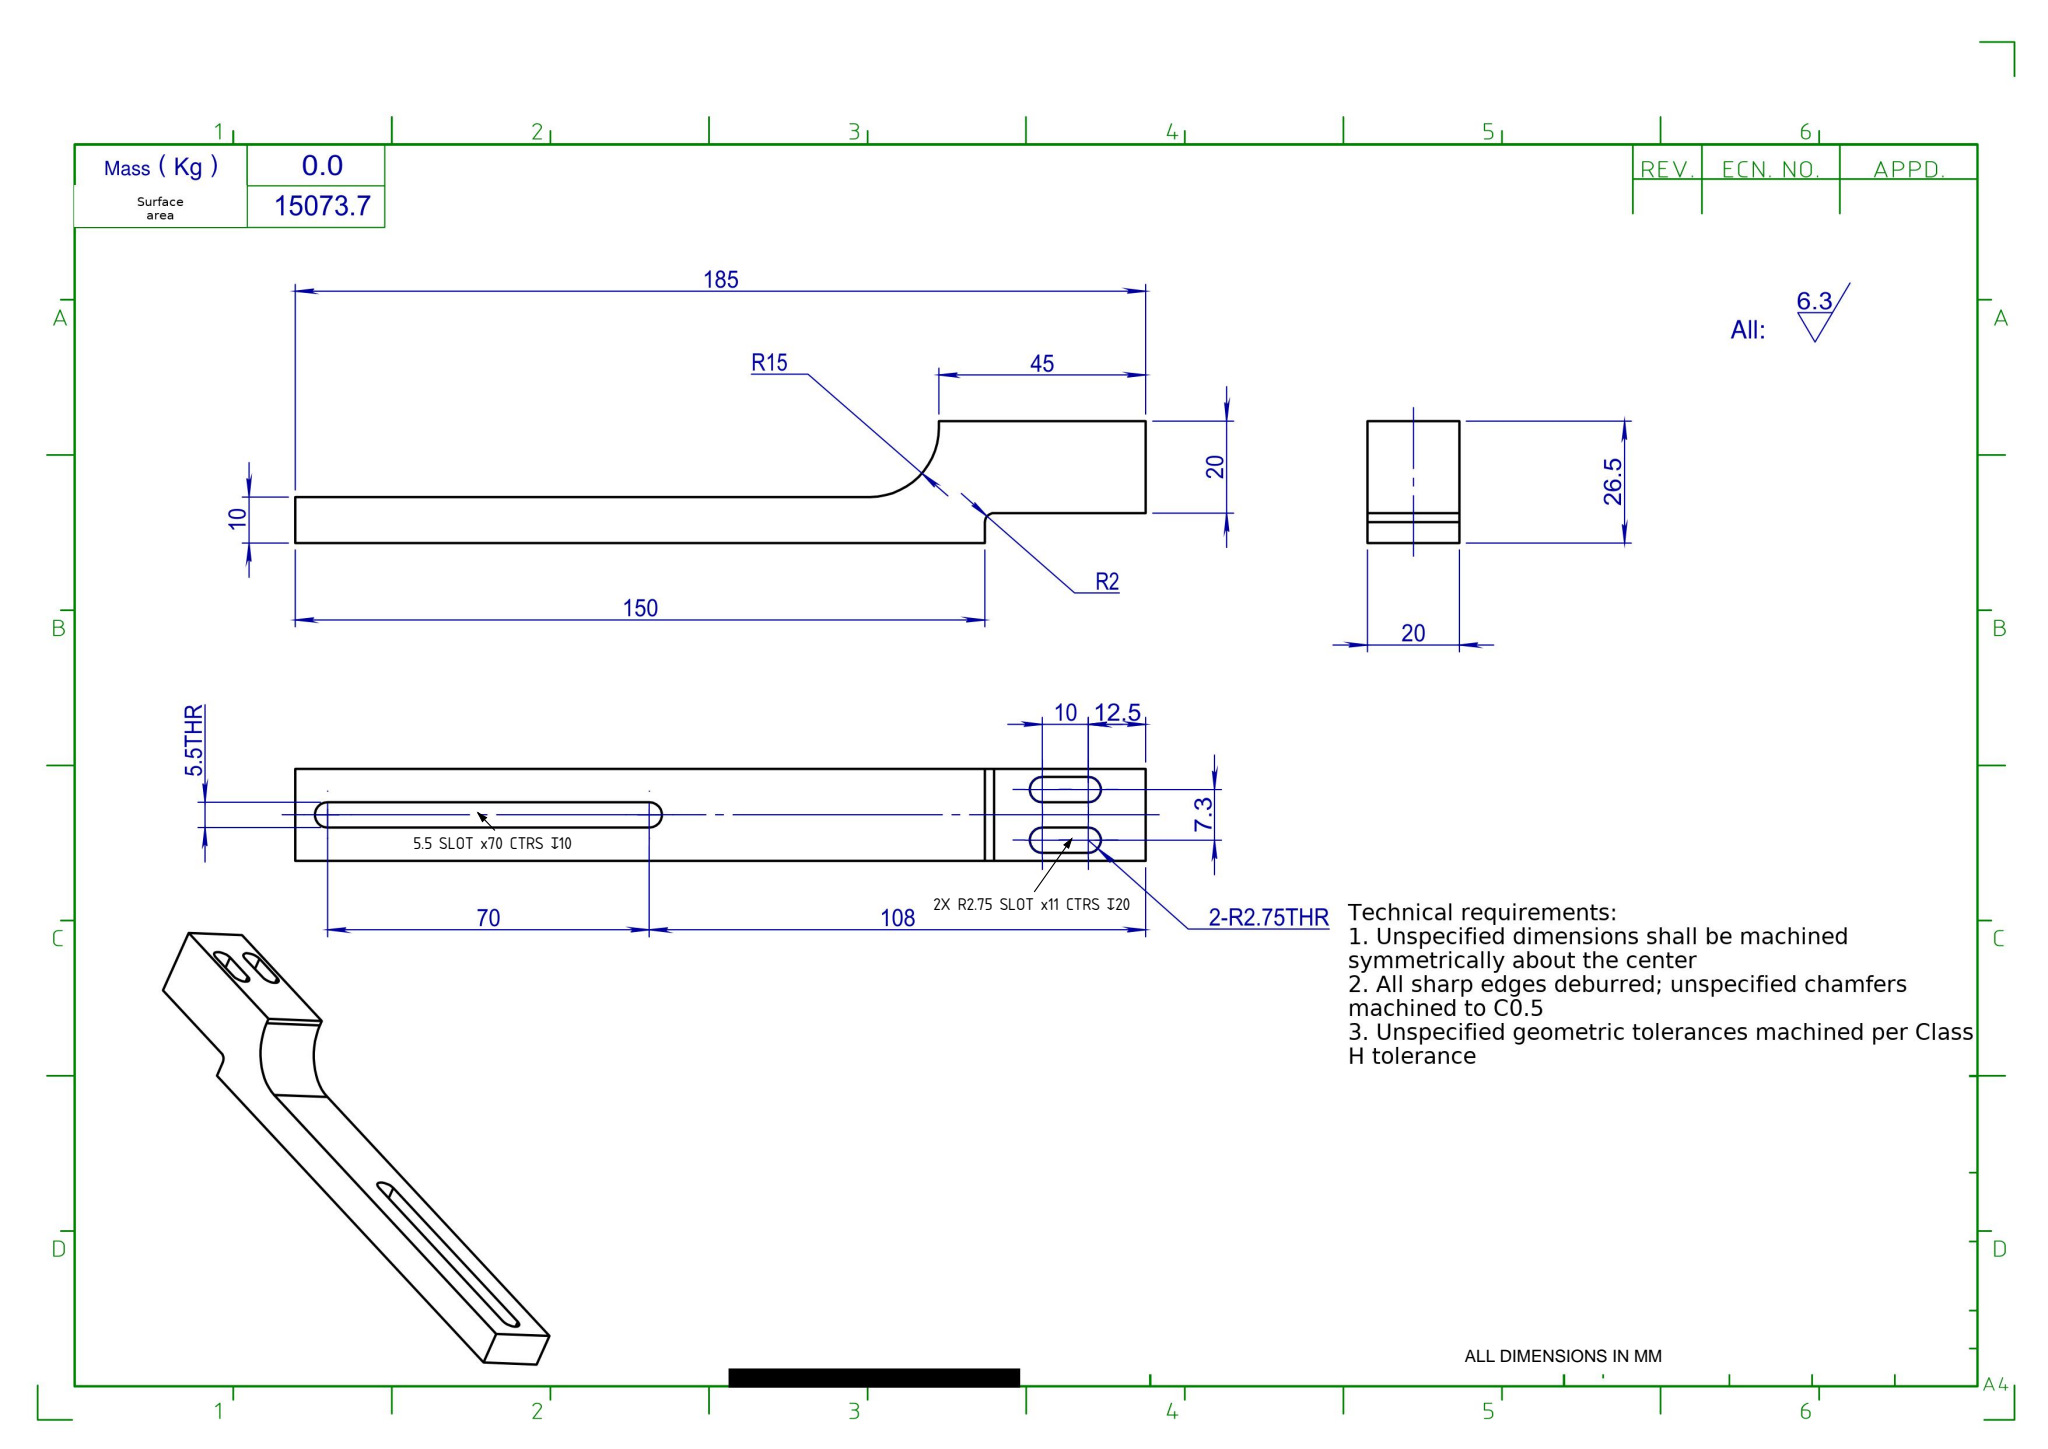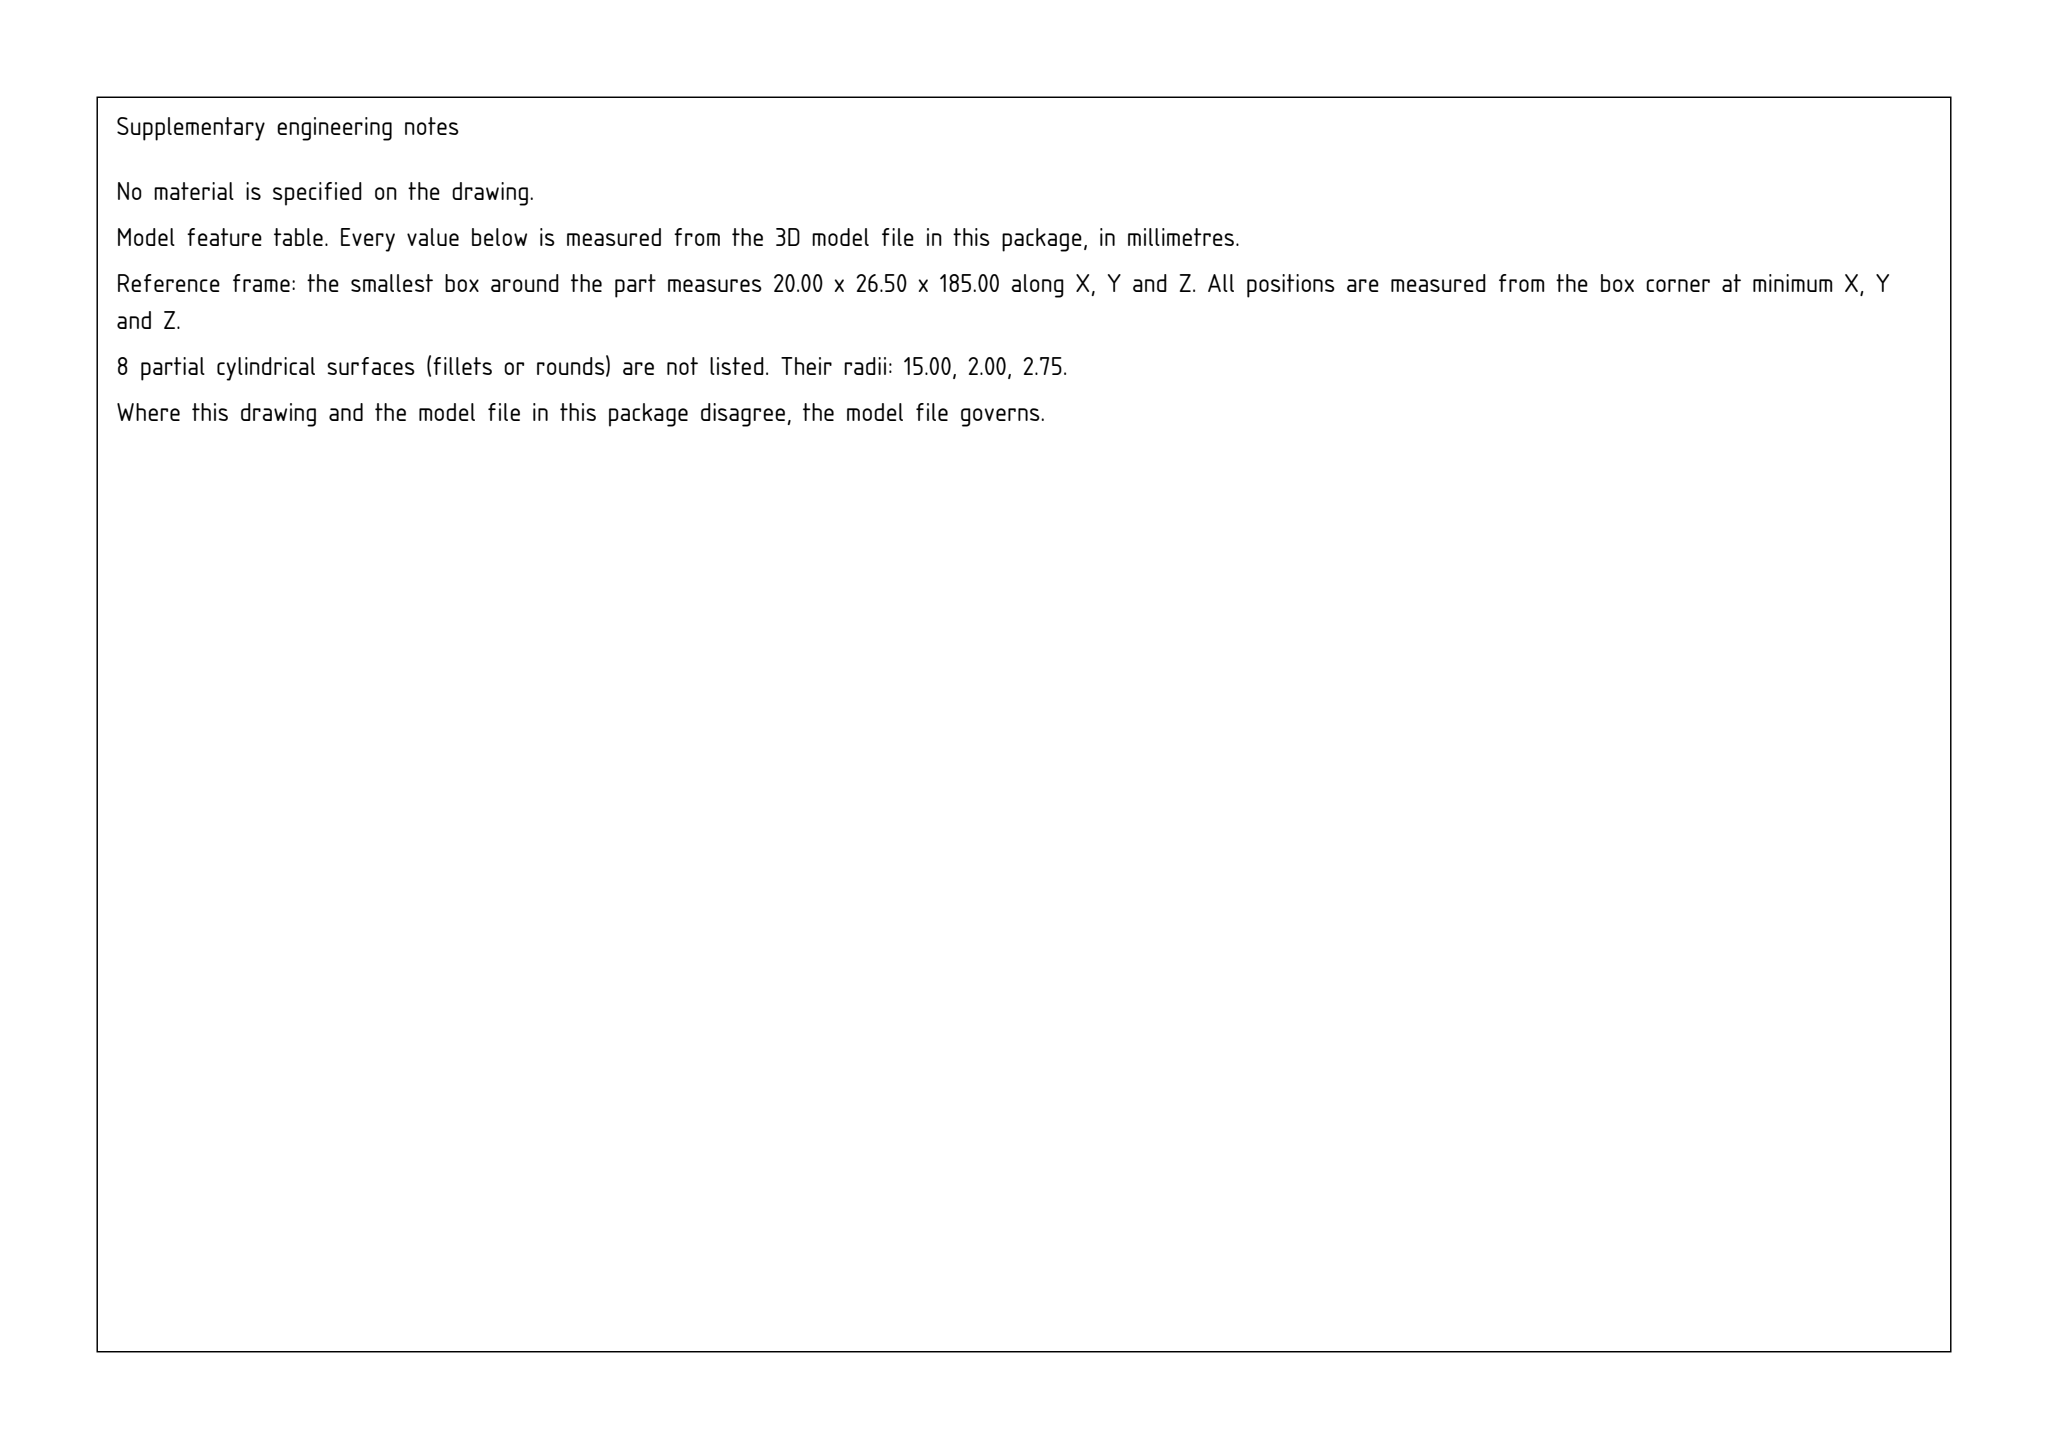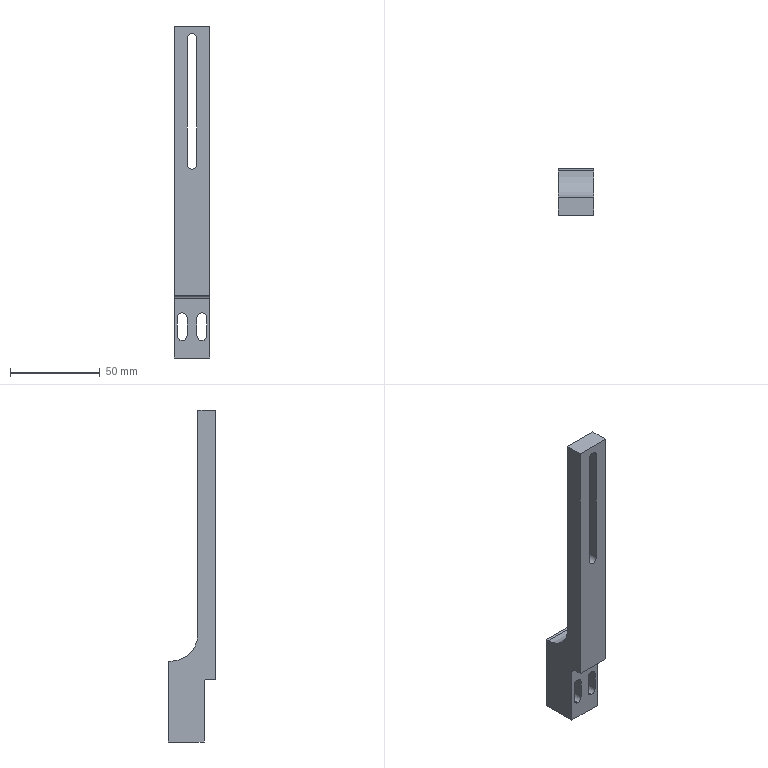Part | SolidWorks | mm | 1 solid | 26 faces | box 20 x 26.5 x 185 mm | volume 41045 mm3 | plane 16 | cylinder 10 | commonest cylinder face diameters 5.5 x8 30 x1 4 x1
Drawing notes:
CTR SLOT 5.5 WIDE x 70 BTWN CTRS, THRU 10 | from the solid: Two d5.5 y-axis arcs at x=10, z=108 & 178, y 0->10; 70 apart
2-R2.75 SLOTS 5.5 WIDE x 11 BTWN CTRS, THRU 20 | from the solid: d5.5 y-axis arcs at x=4.5 & 15.5, z=12.5 & 22.5, y 6.5->26.5
build123d program:
from build123d import *

# Parameters (mm, degrees)
SKETCH1_W           = 20
SKETCH1_H           = 10
BOSS_EXTRUDE1_DEPTH = 150
SKETCH2_W           = 20
SKETCH2_H           = 10
BOSS_EXTRUDE2_DEPTH = 16.5
CUT_EXTRUDE2_DEPTH  = 153.651
FILLET1_R           = 15
SKETCH12_W          = 20
SKETCH12_H          = 20
BOSS_EXTRUDE3_DEPTH = 35
CUT_EXTRUDE3_DEPTH  = 152.658
FILLET2_R           = 2


with BuildPart() as part:
    # Sketch1 → Boss-Extrude1 (new body)
    with BuildSketch(Plane.XY):
        Rectangle(SKETCH1_W, SKETCH1_H)
    extrude(amount=BOSS_EXTRUDE1_DEPTH)

    # Sketch2 → Boss-Extrude2 (add)
    with BuildSketch(Plane(origin=(0, 5, 0), x_dir=(1, 0, 0), z_dir=(0, 1, 0))):
        with Locations((0, -5)):
            Rectangle(SKETCH2_W, SKETCH2_H)
    extrude(amount=BOSS_EXTRUDE2_DEPTH)

    # Sketch9 → Cut-Extrude2 (cut, through all)
    with BuildSketch(Plane.XZ.offset(5)):
        with BuildLine():
            Line((-2.75, 143), (-2.75, 73))
            ThreePointArc((-2.75, 73), (0, 70.25), (2.75, 73))
            Line((2.75, 73), (2.75, 143))
            ThreePointArc((2.75, 143), (0, 145.75), (-2.75, 143))
        make_face()
    extrude(amount=-CUT_EXTRUDE2_DEPTH, mode=Mode.SUBTRACT)

    # Fillet1
    fillet1_edges = [part.edges().sort_by_distance(p)[0] for p in [
        (0, 5, 10),
    ]]
    fillet(fillet1_edges, radius=FILLET1_R)

    # Sketch12 → Boss-Extrude3 (add)
    with BuildSketch(Plane(origin=(0, 0, 0), x_dir=(-1, 0, 0), z_dir=(0, 0, -1))):
        with Locations((0, 11.5)):
            Rectangle(SKETCH12_W, SKETCH12_H)
    extrude(amount=BOSS_EXTRUDE3_DEPTH)

    # Sketch13 → Cut-Extrude3 (cut, through all)
    with BuildSketch(Plane.XZ.offset(-1.5)):
        with BuildLine():
            Line((-8.25, -22.5), (-8.25, -12.5))
            ThreePointArc((-8.25, -12.5), (-5.5, -9.75), (-2.75, -12.5))
            Line((-2.75, -12.5), (-2.75, -22.5))
            ThreePointArc((-2.75, -22.5), (-5.5, -25.25), (-8.25, -22.5))
        make_face()
        with BuildLine():
            Line((8.25, -22.5), (8.25, -12.5))
            ThreePointArc((8.25, -12.5), (5.5, -9.75), (2.75, -12.5))
            Line((2.75, -12.5), (2.75, -22.5))
            ThreePointArc((2.75, -22.5), (5.5, -25.25), (8.25, -22.5))
        make_face()
    extrude(amount=-CUT_EXTRUDE3_DEPTH, mode=Mode.SUBTRACT)

    # Fillet2
    fillet2_edges = [part.edges().sort_by_distance(p)[0] for p in [
        (0, 1.5, 0),
    ]]
    fillet(fillet2_edges, radius=FILLET2_R)


solid = part.part
STEP:
#1=CARTESIAN_POINT('',(5.5,21.5,-25.25));
#2=VERTEX_POINT('',#1);
#3=CARTESIAN_POINT('',(8.25,21.5,-22.5));
#4=VERTEX_POINT('',#3);
#5=CARTESIAN_POINT('',(5.5,21.5,-22.5));
#6=DIRECTION('',(0.,-1.,0.));
#7=DIRECTION('',(0.,0.,1.));
#8=AXIS2_PLACEMENT_3D('',#5,#6,#7);
#9=CIRCLE('',#8,2.75);
#10=EDGE_CURVE('',#2,#4,#9,.T.);
#11=ORIENTED_EDGE('',*,*,#10,.F.);
#12=CARTESIAN_POINT('',(5.5,1.5,-25.25));
#13=VERTEX_POINT('',#12);
#14=CARTESIAN_POINT('',(5.5,21.5,-25.25));
#15=DIRECTION('',(0.,-1.,0.));
#16=VECTOR('',#15,1000.);
#17=LINE('',#14,#16);
#18=EDGE_CURVE('',#2,#13,#17,.T.);
#19=ORIENTED_EDGE('',*,*,#18,.T.);
#20=CARTESIAN_POINT('',(8.25,1.5,-22.5));
#21=VERTEX_POINT('',#20);
#22=CARTESIAN_POINT('',(5.5,1.5,-22.5));
#23=DIRECTION('',(0.,-1.,0.));
#24=DIRECTION('',(0.,0.,1.));
#25=AXIS2_PLACEMENT_3D('',#22,#23,#24);
#26=CIRCLE('',#25,2.75);
#27=EDGE_CURVE('',#13,#21,#26,.T.);
#28=ORIENTED_EDGE('',*,*,#27,.T.);
#29=CARTESIAN_POINT('',(8.25,21.5,-22.5));
#30=DIRECTION('',(0.,-1.,0.));
#31=VECTOR('',#30,1000.);
#32=LINE('',#29,#31);
#33=EDGE_CURVE('',#4,#21,#32,.T.);
#34=ORIENTED_EDGE('',*,*,#33,.F.);
#35=EDGE_LOOP('',(#11,#19,#28,#34));
#36=FACE_OUTER_BOUND('',#35,.T.);
#37=CARTESIAN_POINT('',(5.5,21.5,-22.5));
#38=DIRECTION('',(0.,-1.,0.));
#39=DIRECTION('',(0.,0.,-1.));
#40=AXIS2_PLACEMENT_3D('',#37,#38,#39);
#41=CYLINDRICAL_SURFACE('',#40,2.75);
#42=ADVANCED_FACE('',(#36),#41,.F.);
#43=CARTESIAN_POINT('',(-5.5,21.5,-25.25));
#44=VERTEX_POINT('',#43);
#45=CARTESIAN_POINT('',(-2.75,21.5,-22.5));
#46=VERTEX_POINT('',#45);
#47=CARTESIAN_POINT('',(-5.5,21.5,-22.5));
#48=DIRECTION('',(0.,-1.,0.));
#49=DIRECTION('',(0.,0.,-1.));
#50=AXIS2_PLACEMENT_3D('',#47,#48,#49);
#51=CIRCLE('',#50,2.75);
#52=EDGE_CURVE('',#44,#46,#51,.T.);
#53=ORIENTED_EDGE('',*,*,#52,.F.);
#54=CARTESIAN_POINT('',(-5.5,1.5,-25.25));
#55=VERTEX_POINT('',#54);
#56=CARTESIAN_POINT('',(-5.5,21.5,-25.25));
#57=DIRECTION('',(0.,-1.,0.));
#58=VECTOR('',#57,1000.);
#59=LINE('',#56,#58);
#60=EDGE_CURVE('',#44,#55,#59,.T.);
#61=ORIENTED_EDGE('',*,*,#60,.T.);
#62=CARTESIAN_POINT('',(-2.75,1.5,-22.5));
#63=VERTEX_POINT('',#62);
#64=CARTESIAN_POINT('',(-5.5,1.5,-22.5));
#65=DIRECTION('',(0.,-1.,0.));
#66=DIRECTION('',(0.,0.,-1.));
#67=AXIS2_PLACEMENT_3D('',#64,#65,#66);
#68=CIRCLE('',#67,2.75);
#69=EDGE_CURVE('',#55,#63,#68,.T.);
#70=ORIENTED_EDGE('',*,*,#69,.T.);
#71=CARTESIAN_POINT('',(-2.75,21.5,-22.5));
#72=DIRECTION('',(0.,-1.,0.));
#73=VECTOR('',#72,1000.);
#74=LINE('',#71,#73);
#75=EDGE_CURVE('',#46,#63,#74,.T.);
#76=ORIENTED_EDGE('',*,*,#75,.F.);
#77=EDGE_LOOP('',(#53,#61,#70,#76));
#78=FACE_OUTER_BOUND('',#77,.T.);
#79=CARTESIAN_POINT('',(-5.5,21.5,-22.5));
#80=DIRECTION('',(0.,-1.,0.));
#81=DIRECTION('',(0.,0.,-1.));
#82=AXIS2_PLACEMENT_3D('',#79,#80,#81);
#83=CYLINDRICAL_SURFACE('',#82,2.75);
#84=ADVANCED_FACE('',(#78),#83,.F.);
#85=CARTESIAN_POINT('',(-10.,-0.5,0.));
#86=VERTEX_POINT('',#85);
#87=CARTESIAN_POINT('',(-10.,-5.,0.));
#88=VERTEX_POINT('',#87);
#89=CARTESIAN_POINT('',(-10.,-5.,0.));
#90=DIRECTION('',(0.,-1.,0.));
#91=VECTOR('',#90,1000.);
#92=LINE('',#89,#91);
#93=EDGE_CURVE('',#86,#88,#92,.T.);
#94=ORIENTED_EDGE('',*,*,#93,.F.);
#95=CARTESIAN_POINT('',(10.,-0.5,0.));
#96=VERTEX_POINT('',#95);
#97=CARTESIAN_POINT('',(10.,-0.5,0.));
#98=DIRECTION('',(1.,0.,0.));
#99=VECTOR('',#98,1000.);
#100=LINE('',#97,#99);
#101=EDGE_CURVE('',#86,#96,#100,.T.);
#102=ORIENTED_EDGE('',*,*,#101,.T.);
#103=CARTESIAN_POINT('',(10.,-5.,0.));
#104=VERTEX_POINT('',#103);
#105=CARTESIAN_POINT('',(10.,-5.,0.));
#106=DIRECTION('',(0.,1.,0.));
#107=VECTOR('',#106,1000.);
#108=LINE('',#105,#107);
#109=EDGE_CURVE('',#104,#96,#108,.T.);
#110=ORIENTED_EDGE('',*,*,#109,.F.);
#111=CARTESIAN_POINT('',(10.,-5.,0.));
#112=DIRECTION('',(1.,0.,0.));
#113=VECTOR('',#112,1000.);
#114=LINE('',#111,#113);
#115=EDGE_CURVE('',#88,#104,#114,.T.);
#116=ORIENTED_EDGE('',*,*,#115,.F.);
#117=EDGE_LOOP('',(#94,#102,#110,#116));
#118=FACE_OUTER_BOUND('',#117,.T.);
#119=CARTESIAN_POINT('',(0.,0.,0.));
#120=DIRECTION('',(0.,0.,1.));
#121=DIRECTION('',(1.,0.,0.));
#122=AXIS2_PLACEMENT_3D('',#119,#120,#121);
#123=PLANE('',#122);
#124=ADVANCED_FACE('',(#118),#123,.F.);
#125=CARTESIAN_POINT('',(2.75,5.,73.));
#126=VERTEX_POINT('',#125);
#127=CARTESIAN_POINT('',(2.75,5.,143.));
#128=VERTEX_POINT('',#127);
#129=CARTESIAN_POINT('',(2.75,5.,150.));
#130=DIRECTION('',(0.,0.,1.));
#131=VECTOR('',#130,1000.);
#132=LINE('',#129,#131);
#133=EDGE_CURVE('',#126,#128,#132,.T.);
#134=ORIENTED_EDGE('',*,*,#133,.T.);
#135=CARTESIAN_POINT('',(-2.75,5.,143.));
#136=VERTEX_POINT('',#135);
#137=CARTESIAN_POINT('',(-0.,5.,143.));
#138=DIRECTION('',(0.,-1.,0.));
#139=DIRECTION('',(1.,0.,0.));
#140=AXIS2_PLACEMENT_3D('',#137,#138,#139);
#141=CIRCLE('',#140,2.75);
#142=EDGE_CURVE('',#128,#136,#141,.T.);
#143=ORIENTED_EDGE('',*,*,#142,.T.);
#144=CARTESIAN_POINT('',(-2.75,5.,73.));
#145=VERTEX_POINT('',#144);
#146=CARTESIAN_POINT('',(-2.75,5.,150.));
#147=DIRECTION('',(0.,0.,-1.));
#148=VECTOR('',#147,1000.);
#149=LINE('',#146,#148);
#150=EDGE_CURVE('',#136,#145,#149,.T.);
#151=ORIENTED_EDGE('',*,*,#150,.T.);
#152=CARTESIAN_POINT('',(0.,5.,73.));
#153=DIRECTION('',(0.,-1.,0.));
#154=DIRECTION('',(1.,0.,0.));
#155=AXIS2_PLACEMENT_3D('',#152,#153,#154);
#156=CIRCLE('',#155,2.75);
#157=EDGE_CURVE('',#145,#126,#156,.T.);
#158=ORIENTED_EDGE('',*,*,#157,.T.);
#159=EDGE_LOOP('',(#134,#143,#151,#158));
#160=FACE_BOUND('',#159,.T.);
#161=CARTESIAN_POINT('',(10.,5.,150.));
#162=VERTEX_POINT('',#161);
#163=CARTESIAN_POINT('',(10.,5.,25.));
#164=VERTEX_POINT('',#163);
#165=CARTESIAN_POINT('',(10.,5.,150.));
#166=DIRECTION('',(0.,0.,-1.));
#167=VECTOR('',#166,1000.);
#168=LINE('',#165,#167);
#169=EDGE_CURVE('',#162,#164,#168,.T.);
#170=ORIENTED_EDGE('',*,*,#169,.T.);
#171=CARTESIAN_POINT('',(-10.,5.,25.));
#172=VERTEX_POINT('',#171);
#173=CARTESIAN_POINT('',(-10.,5.,25.));
#174=DIRECTION('',(-1.,-0.,-0.));
#175=VECTOR('',#174,1000.);
#176=LINE('',#173,#175);
#177=EDGE_CURVE('',#164,#172,#176,.T.);
#178=ORIENTED_EDGE('',*,*,#177,.T.);
#179=CARTESIAN_POINT('',(-10.,5.,150.));
#180=VERTEX_POINT('',#179);
#181=CARTESIAN_POINT('',(-10.,5.,150.));
#182=DIRECTION('',(0.,0.,-1.));
#183=VECTOR('',#182,1000.);
#184=LINE('',#181,#183);
#185=EDGE_CURVE('',#180,#172,#184,.T.);
#186=ORIENTED_EDGE('',*,*,#185,.F.);
#187=CARTESIAN_POINT('',(10.,5.,150.));
#188=DIRECTION('',(-1.,-0.,0.));
#189=VECTOR('',#188,1000.);
#190=LINE('',#187,#189);
#191=EDGE_CURVE('',#162,#180,#190,.T.);
#192=ORIENTED_EDGE('',*,*,#191,.F.);
#193=EDGE_LOOP('',(#170,#178,#186,#192));
#194=FACE_OUTER_BOUND('',#193,.T.);
#195=CARTESIAN_POINT('',(10.,5.,150.));
#196=DIRECTION('',(0.,-1.,0.));
#197=DIRECTION('',(1.,0.,0.));
#198=AXIS2_PLACEMENT_3D('',#195,#196,#197);
#199=PLANE('',#198);
#200=ADVANCED_FACE('',(#160,#194),#199,.F.);
#201=CARTESIAN_POINT('',(-10.,21.5,-35.));
#202=VERTEX_POINT('',#201);
#203=CARTESIAN_POINT('',(-10.,21.5,10.));
#204=VERTEX_POINT('',#203);
#205=CARTESIAN_POINT('',(-10.,21.5,0.));
#206=DIRECTION('',(0.,0.,1.));
#207=VECTOR('',#206,1000.);
#208=LINE('',#205,#207);
#209=EDGE_CURVE('',#202,#204,#208,.T.);
#210=ORIENTED_EDGE('',*,*,#209,.F.);
#211=CARTESIAN_POINT('',(-10.,1.5,-35.));
#212=VERTEX_POINT('',#211);
#213=CARTESIAN_POINT('',(-10.,21.5,-35.));
#214=DIRECTION('',(0.,1.,0.));
#215=VECTOR('',#214,1000.);
#216=LINE('',#213,#215);
#217=EDGE_CURVE('',#212,#202,#216,.T.);
#218=ORIENTED_EDGE('',*,*,#217,.F.);
#219=CARTESIAN_POINT('',(-10.,1.5,-2.));
#220=VERTEX_POINT('',#219);
#221=CARTESIAN_POINT('',(-10.,1.5,-35.));
#222=DIRECTION('',(0.,0.,1.));
#223=VECTOR('',#222,1000.);
#224=LINE('',#221,#223);
#225=EDGE_CURVE('',#212,#220,#224,.T.);
#226=ORIENTED_EDGE('',*,*,#225,.T.);
#227=CARTESIAN_POINT('',(-10.,-0.5,-2.));
#228=DIRECTION('',(1.,0.,0.));
#229=DIRECTION('',(0.,0.,-1.));
#230=AXIS2_PLACEMENT_3D('',#227,#228,#229);
#231=CIRCLE('',#230,2.);
#232=EDGE_CURVE('',#220,#86,#231,.T.);
#233=ORIENTED_EDGE('',*,*,#232,.T.);
#234=ORIENTED_EDGE('',*,*,#93,.T.);
#235=CARTESIAN_POINT('',(-10.,-5.,150.));
#236=VERTEX_POINT('',#235);
#237=CARTESIAN_POINT('',(-10.,-5.,150.));
#238=DIRECTION('',(0.,0.,-1.));
#239=VECTOR('',#238,1000.);
#240=LINE('',#237,#239);
#241=EDGE_CURVE('',#236,#88,#240,.T.);
#242=ORIENTED_EDGE('',*,*,#241,.F.);
#243=CARTESIAN_POINT('',(-10.,-5.,150.));
#244=DIRECTION('',(0.,-1.,0.));
#245=VECTOR('',#244,1000.);
#246=LINE('',#243,#245);
#247=EDGE_CURVE('',#180,#236,#246,.T.);
#248=ORIENTED_EDGE('',*,*,#247,.F.);
#249=ORIENTED_EDGE('',*,*,#185,.T.);
#250=CARTESIAN_POINT('',(-10.,20.,10.));
#251=VERTEX_POINT('',#250);
#252=CARTESIAN_POINT('',(-10.,20.,25.));
#253=DIRECTION('',(1.,0.,0.));
#254=DIRECTION('',(0.,0.,-1.));
#255=AXIS2_PLACEMENT_3D('',#252,#253,#254);
#256=CIRCLE('',#255,15.);
#257=EDGE_CURVE('',#172,#251,#256,.T.);
#258=ORIENTED_EDGE('',*,*,#257,.T.);
#259=CARTESIAN_POINT('',(-10.,21.5,10.));
#260=DIRECTION('',(0.,-1.,0.));
#261=VECTOR('',#260,1000.);
#262=LINE('',#259,#261);
#263=EDGE_CURVE('',#204,#251,#262,.T.);
#264=ORIENTED_EDGE('',*,*,#263,.F.);
#265=EDGE_LOOP('',(#210,#218,#226,#233,#234,#242,#248,#249,#258,#264));
#266=FACE_OUTER_BOUND('',#265,.T.);
#267=CARTESIAN_POINT('',(-10.,-5.,150.));
#268=DIRECTION('',(1.,0.,0.));
#269=DIRECTION('',(0.,0.,-1.));
#270=AXIS2_PLACEMENT_3D('',#267,#268,#269);
#271=PLANE('',#270);
#272=ADVANCED_FACE('',(#266),#271,.F.);
#273=CARTESIAN_POINT('',(-2.75,-5.,143.));
#274=VERTEX_POINT('',#273);
#275=CARTESIAN_POINT('',(-2.75,-5.,73.));
#276=VERTEX_POINT('',#275);
#277=CARTESIAN_POINT('',(-2.75,-5.,143.));
#278=DIRECTION('',(0.,0.,-1.));
#279=VECTOR('',#278,1000.);
#280=LINE('',#277,#279);
#281=EDGE_CURVE('',#274,#276,#280,.T.);
#282=ORIENTED_EDGE('',*,*,#281,.F.);
#283=CARTESIAN_POINT('',(2.75,-5.,143.));
#284=VERTEX_POINT('',#283);
#285=CARTESIAN_POINT('',(0.,-5.,143.));
#286=DIRECTION('',(0.,-1.,0.));
#287=DIRECTION('',(1.,0.,0.));
#288=AXIS2_PLACEMENT_3D('',#285,#286,#287);
#289=CIRCLE('',#288,2.75);
#290=EDGE_CURVE('',#284,#274,#289,.T.);
#291=ORIENTED_EDGE('',*,*,#290,.F.);
#292=CARTESIAN_POINT('',(2.75,-5.,73.));
#293=VERTEX_POINT('',#292);
#294=CARTESIAN_POINT('',(2.75,-5.,143.));
#295=DIRECTION('',(0.,0.,1.));
#296=VECTOR('',#295,1000.);
#297=LINE('',#294,#296);
#298=EDGE_CURVE('',#293,#284,#297,.T.);
#299=ORIENTED_EDGE('',*,*,#298,.F.);
#300=CARTESIAN_POINT('',(0.,-5.,73.));
#301=DIRECTION('',(0.,-1.,0.));
#302=DIRECTION('',(1.,0.,0.));
#303=AXIS2_PLACEMENT_3D('',#300,#301,#302);
#304=CIRCLE('',#303,2.75);
#305=EDGE_CURVE('',#276,#293,#304,.T.);
#306=ORIENTED_EDGE('',*,*,#305,.F.);
#307=EDGE_LOOP('',(#282,#291,#299,#306));
#308=FACE_BOUND('',#307,.T.);
#309=ORIENTED_EDGE('',*,*,#115,.T.);
#310=CARTESIAN_POINT('',(10.,-5.,150.));
#311=VERTEX_POINT('',#310);
#312=CARTESIAN_POINT('',(10.,-5.,150.));
#313=DIRECTION('',(0.,0.,-1.));
#314=VECTOR('',#313,1000.);
#315=LINE('',#312,#314);
#316=EDGE_CURVE('',#311,#104,#315,.T.);
#317=ORIENTED_EDGE('',*,*,#316,.F.);
#318=CARTESIAN_POINT('',(10.,-5.,150.));
#319=DIRECTION('',(1.,0.,0.));
#320=VECTOR('',#319,1000.);
#321=LINE('',#318,#320);
#322=EDGE_CURVE('',#236,#311,#321,.T.);
#323=ORIENTED_EDGE('',*,*,#322,.F.);
#324=ORIENTED_EDGE('',*,*,#241,.T.);
#325=EDGE_LOOP('',(#309,#317,#323,#324));
#326=FACE_OUTER_BOUND('',#325,.T.);
#327=CARTESIAN_POINT('',(10.,-5.,150.));
#328=DIRECTION('',(-0.,1.,0.));
#329=DIRECTION('',(-1.,-0.,0.));
#330=AXIS2_PLACEMENT_3D('',#327,#328,#329);
#331=PLANE('',#330);
#332=ADVANCED_FACE('',(#308,#326),#331,.F.);
#333=ORIENTED_EDGE('',*,*,#109,.T.);
#334=CARTESIAN_POINT('',(10.,1.5,-2.));
#335=VERTEX_POINT('',#334);
#336=CARTESIAN_POINT('',(10.,-0.5,-2.));
#337=DIRECTION('',(-1.,0.,0.));
#338=DIRECTION('',(0.,0.,1.));
#339=AXIS2_PLACEMENT_3D('',#336,#337,#338);
#340=CIRCLE('',#339,2.);
#341=EDGE_CURVE('',#96,#335,#340,.T.);
#342=ORIENTED_EDGE('',*,*,#341,.T.);
#343=CARTESIAN_POINT('',(10.,1.5,-35.));
#344=VERTEX_POINT('',#343);
#345=CARTESIAN_POINT('',(10.,1.5,-35.));
#346=DIRECTION('',(0.,0.,1.));
#347=VECTOR('',#346,1000.);
#348=LINE('',#345,#347);
#349=EDGE_CURVE('',#344,#335,#348,.T.);
#350=ORIENTED_EDGE('',*,*,#349,.F.);
#351=CARTESIAN_POINT('',(10.,21.5,-35.));
#352=VERTEX_POINT('',#351);
#353=CARTESIAN_POINT('',(10.,21.5,-35.));
#354=DIRECTION('',(-0.,-1.,0.));
#355=VECTOR('',#354,1000.);
#356=LINE('',#353,#355);
#357=EDGE_CURVE('',#352,#344,#356,.T.);
#358=ORIENTED_EDGE('',*,*,#357,.F.);
#359=CARTESIAN_POINT('',(10.,21.5,10.));
#360=VERTEX_POINT('',#359);
#361=CARTESIAN_POINT('',(10.,21.5,0.));
#362=DIRECTION('',(0.,0.,-1.));
#363=VECTOR('',#362,1000.);
#364=LINE('',#361,#363);
#365=EDGE_CURVE('',#360,#352,#364,.T.);
#366=ORIENTED_EDGE('',*,*,#365,.F.);
#367=CARTESIAN_POINT('',(10.,20.,10.));
#368=VERTEX_POINT('',#367);
#369=CARTESIAN_POINT('',(10.,21.5,10.));
#370=DIRECTION('',(0.,-1.,0.));
#371=VECTOR('',#370,1000.);
#372=LINE('',#369,#371);
#373=EDGE_CURVE('',#360,#368,#372,.T.);
#374=ORIENTED_EDGE('',*,*,#373,.T.);
#375=CARTESIAN_POINT('',(10.,20.,25.));
#376=DIRECTION('',(-1.,0.,0.));
#377=DIRECTION('',(0.,0.,1.));
#378=AXIS2_PLACEMENT_3D('',#375,#376,#377);
#379=CIRCLE('',#378,15.);
#380=EDGE_CURVE('',#368,#164,#379,.T.);
#381=ORIENTED_EDGE('',*,*,#380,.T.);
#382=ORIENTED_EDGE('',*,*,#169,.F.);
#383=CARTESIAN_POINT('',(10.,-5.,150.));
#384=DIRECTION('',(0.,1.,0.));
#385=VECTOR('',#384,1000.);
#386=LINE('',#383,#385);
#387=EDGE_CURVE('',#311,#162,#386,.T.);
#388=ORIENTED_EDGE('',*,*,#387,.F.);
#389=ORIENTED_EDGE('',*,*,#316,.T.);
#390=EDGE_LOOP('',(#333,#342,#350,#358,#366,#374,#381,#382,#388,#389));
#391=FACE_OUTER_BOUND('',#390,.T.);
#392=CARTESIAN_POINT('',(10.,-5.,150.));
#393=DIRECTION('',(-1.,0.,0.));
#394=DIRECTION('',(0.,0.,1.));
#395=AXIS2_PLACEMENT_3D('',#392,#393,#394);
#396=PLANE('',#395);
#397=ADVANCED_FACE('',(#391),#396,.F.);
#398=ORIENTED_EDGE('',*,*,#247,.T.);
#399=ORIENTED_EDGE('',*,*,#322,.T.);
#400=ORIENTED_EDGE('',*,*,#387,.T.);
#401=ORIENTED_EDGE('',*,*,#191,.T.);
#402=EDGE_LOOP('',(#398,#399,#400,#401));
#403=FACE_OUTER_BOUND('',#402,.T.);
#404=CARTESIAN_POINT('',(0.,0.,150.));
#405=DIRECTION('',(0.,0.,1.));
#406=DIRECTION('',(1.,0.,0.));
#407=AXIS2_PLACEMENT_3D('',#404,#405,#406);
#408=PLANE('',#407);
#409=ADVANCED_FACE('',(#403),#408,.T.);
#410=ORIENTED_EDGE('',*,*,#263,.T.);
#411=CARTESIAN_POINT('',(10.,20.,10.));
#412=DIRECTION('',(1.,0.,0.));
#413=VECTOR('',#412,1000.);
#414=LINE('',#411,#413);
#415=EDGE_CURVE('',#251,#368,#414,.T.);
#416=ORIENTED_EDGE('',*,*,#415,.T.);
#417=ORIENTED_EDGE('',*,*,#373,.F.);
#418=CARTESIAN_POINT('',(-10.,21.5,10.));
#419=DIRECTION('',(1.,0.,0.));
#420=VECTOR('',#419,1000.);
#421=LINE('',#418,#420);
#422=EDGE_CURVE('',#204,#360,#421,.T.);
#423=ORIENTED_EDGE('',*,*,#422,.F.);
#424=EDGE_LOOP('',(#410,#416,#417,#423));
#425=FACE_OUTER_BOUND('',#424,.T.);
#426=CARTESIAN_POINT('',(-10.,21.5,10.));
#427=DIRECTION('',(0.,0.,-1.));
#428=DIRECTION('',(-1.,0.,-0.));
#429=AXIS2_PLACEMENT_3D('',#426,#427,#428);
#430=PLANE('',#429);
#431=ADVANCED_FACE('',(#425),#430,.F.);
#432=CARTESIAN_POINT('',(2.75,21.5,-22.5));
#433=VERTEX_POINT('',#432);
#434=CARTESIAN_POINT('',(5.5,21.5,-22.5));
#435=DIRECTION('',(0.,-1.,0.));
#436=DIRECTION('',(0.,0.,1.));
#437=AXIS2_PLACEMENT_3D('',#434,#435,#436);
#438=CIRCLE('',#437,2.75);
#439=EDGE_CURVE('',#433,#2,#438,.T.);
#440=ORIENTED_EDGE('',*,*,#439,.T.);
#441=ORIENTED_EDGE('',*,*,#10,.T.);
#442=CARTESIAN_POINT('',(8.25,21.5,-12.5));
#443=VERTEX_POINT('',#442);
#444=CARTESIAN_POINT('',(8.25,21.5,-22.5));
#445=DIRECTION('',(-0.,0.,1.));
#446=VECTOR('',#445,1000.);
#447=LINE('',#444,#446);
#448=EDGE_CURVE('',#4,#443,#447,.T.);
#449=ORIENTED_EDGE('',*,*,#448,.T.);
#450=CARTESIAN_POINT('',(2.75,21.5,-12.5));
#451=VERTEX_POINT('',#450);
#452=CARTESIAN_POINT('',(5.5,21.5,-12.5));
#453=DIRECTION('',(0.,-1.,0.));
#454=DIRECTION('',(0.,0.,1.));
#455=AXIS2_PLACEMENT_3D('',#452,#453,#454);
#456=CIRCLE('',#455,2.75);
#457=EDGE_CURVE('',#443,#451,#456,.T.);
#458=ORIENTED_EDGE('',*,*,#457,.T.);
#459=CARTESIAN_POINT('',(2.75,21.5,-22.5));
#460=DIRECTION('',(0.,0.,-1.));
#461=VECTOR('',#460,1000.);
#462=LINE('',#459,#461);
#463=EDGE_CURVE('',#451,#433,#462,.T.);
#464=ORIENTED_EDGE('',*,*,#463,.T.);
#465=EDGE_LOOP('',(#440,#441,#449,#458,#464));
#466=FACE_BOUND('',#465,.T.);
#467=CARTESIAN_POINT('',(-8.25,21.5,-22.5));
#468=VERTEX_POINT('',#467);
#469=CARTESIAN_POINT('',(-5.5,21.5,-22.5));
#470=DIRECTION('',(0.,-1.,0.));
#471=DIRECTION('',(0.,0.,-1.));
#472=AXIS2_PLACEMENT_3D('',#469,#470,#471);
#473=CIRCLE('',#472,2.75);
#474=EDGE_CURVE('',#468,#44,#473,.T.);
#475=ORIENTED_EDGE('',*,*,#474,.T.);
#476=ORIENTED_EDGE('',*,*,#52,.T.);
#477=CARTESIAN_POINT('',(-2.75,21.5,-12.5));
#478=VERTEX_POINT('',#477);
#479=CARTESIAN_POINT('',(-2.75,21.5,-22.5));
#480=DIRECTION('',(-0.,0.,1.));
#481=VECTOR('',#480,1000.);
#482=LINE('',#479,#481);
#483=EDGE_CURVE('',#46,#478,#482,.T.);
#484=ORIENTED_EDGE('',*,*,#483,.T.);
#485=CARTESIAN_POINT('',(-8.25,21.5,-12.5));
#486=VERTEX_POINT('',#485);
#487=CARTESIAN_POINT('',(-5.5,21.5,-12.5));
#488=DIRECTION('',(0.,-1.,0.));
#489=DIRECTION('',(0.,0.,-1.));
#490=AXIS2_PLACEMENT_3D('',#487,#488,#489);
#491=CIRCLE('',#490,2.75);
#492=EDGE_CURVE('',#478,#486,#491,.T.);
#493=ORIENTED_EDGE('',*,*,#492,.T.);
#494=CARTESIAN_POINT('',(-8.25,21.5,-22.5));
#495=DIRECTION('',(0.,0.,-1.));
#496=VECTOR('',#495,1000.);
#497=LINE('',#494,#496);
#498=EDGE_CURVE('',#486,#468,#497,.T.);
#499=ORIENTED_EDGE('',*,*,#498,.T.);
#500=EDGE_LOOP('',(#475,#476,#484,#493,#499));
#501=FACE_BOUND('',#500,.T.);
#502=ORIENTED_EDGE('',*,*,#209,.T.);
#503=ORIENTED_EDGE('',*,*,#422,.T.);
#504=ORIENTED_EDGE('',*,*,#365,.T.);
#505=CARTESIAN_POINT('',(10.,21.5,-35.));
#506=DIRECTION('',(1.,0.,0.));
#507=VECTOR('',#506,1000.);
#508=LINE('',#505,#507);
#509=EDGE_CURVE('',#202,#352,#508,.T.);
#510=ORIENTED_EDGE('',*,*,#509,.F.);
#511=EDGE_LOOP('',(#502,#503,#504,#510));
#512=FACE_OUTER_BOUND('',#511,.T.);
#513=CARTESIAN_POINT('',(-0.,21.5,0.));
#514=DIRECTION('',(-0.,1.,0.));
#515=DIRECTION('',(-1.,-0.,0.));
#516=AXIS2_PLACEMENT_3D('',#513,#514,#515);
#517=PLANE('',#516);
#518=ADVANCED_FACE('',(#466,#501,#512),#517,.T.);
#519=CARTESIAN_POINT('',(2.75,21.5,143.));
#520=DIRECTION('',(0.,-1.,0.));
#521=VECTOR('',#520,1000.);
#522=LINE('',#519,#521);
#523=EDGE_CURVE('',#128,#284,#522,.T.);
#524=ORIENTED_EDGE('',*,*,#523,.T.);
#525=ORIENTED_EDGE('',*,*,#290,.T.);
#526=CARTESIAN_POINT('',(-2.75,21.5,143.));
#527=DIRECTION('',(0.,-1.,0.));
#528=VECTOR('',#527,1000.);
#529=LINE('',#526,#528);
#530=EDGE_CURVE('',#136,#274,#529,.T.);
#531=ORIENTED_EDGE('',*,*,#530,.F.);
#532=ORIENTED_EDGE('',*,*,#142,.F.);
#533=EDGE_LOOP('',(#524,#525,#531,#532));
#534=FACE_OUTER_BOUND('',#533,.T.);
#535=CARTESIAN_POINT('',(-0.,21.5,143.));
#536=DIRECTION('',(0.,-1.,0.));
#537=DIRECTION('',(1.,0.,0.));
#538=AXIS2_PLACEMENT_3D('',#535,#536,#537);
#539=CYLINDRICAL_SURFACE('',#538,2.75);
#540=ADVANCED_FACE('',(#534),#539,.F.);
#541=CARTESIAN_POINT('',(2.75,21.5,73.));
#542=DIRECTION('',(0.,-1.,0.));
#543=VECTOR('',#542,1000.);
#544=LINE('',#541,#543);
#545=EDGE_CURVE('',#126,#293,#544,.T.);
#546=ORIENTED_EDGE('',*,*,#545,.T.);
#547=ORIENTED_EDGE('',*,*,#298,.T.);
#548=ORIENTED_EDGE('',*,*,#523,.F.);
#549=ORIENTED_EDGE('',*,*,#133,.F.);
#550=EDGE_LOOP('',(#546,#547,#548,#549));
#551=FACE_OUTER_BOUND('',#550,.T.);
#552=CARTESIAN_POINT('',(2.75,21.5,143.));
#553=DIRECTION('',(1.,0.,-0.));
#554=DIRECTION('',(-0.,0.,-1.));
#555=AXIS2_PLACEMENT_3D('',#552,#553,#554);
#556=PLANE('',#555);
#557=ADVANCED_FACE('',(#551),#556,.F.);
#558=CARTESIAN_POINT('',(-2.75,21.5,73.));
#559=DIRECTION('',(0.,-1.,0.));
#560=VECTOR('',#559,1000.);
#561=LINE('',#558,#560);
#562=EDGE_CURVE('',#145,#276,#561,.T.);
#563=ORIENTED_EDGE('',*,*,#562,.T.);
#564=ORIENTED_EDGE('',*,*,#305,.T.);
#565=ORIENTED_EDGE('',*,*,#545,.F.);
#566=ORIENTED_EDGE('',*,*,#157,.F.);
#567=EDGE_LOOP('',(#563,#564,#565,#566));
#568=FACE_OUTER_BOUND('',#567,.T.);
#569=CARTESIAN_POINT('',(0.,21.5,73.));
#570=DIRECTION('',(0.,-1.,0.));
#571=DIRECTION('',(1.,0.,0.));
#572=AXIS2_PLACEMENT_3D('',#569,#570,#571);
#573=CYLINDRICAL_SURFACE('',#572,2.75);
#574=ADVANCED_FACE('',(#568),#573,.F.);
#575=ORIENTED_EDGE('',*,*,#530,.T.);
#576=ORIENTED_EDGE('',*,*,#281,.T.);
#577=ORIENTED_EDGE('',*,*,#562,.F.);
#578=ORIENTED_EDGE('',*,*,#150,.F.);
#579=EDGE_LOOP('',(#575,#576,#577,#578));
#580=FACE_OUTER_BOUND('',#579,.T.);
#581=CARTESIAN_POINT('',(-2.75,21.5,143.));
#582=DIRECTION('',(-1.,-0.,-0.));
#583=DIRECTION('',(-0.,0.,1.));
#584=AXIS2_PLACEMENT_3D('',#581,#582,#583);
#585=PLANE('',#584);
#586=ADVANCED_FACE('',(#580),#585,.F.);
#587=ORIENTED_EDGE('',*,*,#257,.F.);
#588=ORIENTED_EDGE('',*,*,#177,.F.);
#589=ORIENTED_EDGE('',*,*,#380,.F.);
#590=ORIENTED_EDGE('',*,*,#415,.F.);
#591=EDGE_LOOP('',(#587,#588,#589,#590));
#592=FACE_OUTER_BOUND('',#591,.T.);
#593=CARTESIAN_POINT('',(-10.,20.,25.));
#594=DIRECTION('',(-1.,-0.,-0.));
#595=DIRECTION('',(-0.,0.,1.));
#596=AXIS2_PLACEMENT_3D('',#593,#594,#595);
#597=CYLINDRICAL_SURFACE('',#596,15.);
#598=ADVANCED_FACE('',(#592),#597,.F.);
#599=CARTESIAN_POINT('',(8.25,1.5,-12.5));
#600=VERTEX_POINT('',#599);
#601=CARTESIAN_POINT('',(8.25,1.5,-22.5));
#602=DIRECTION('',(-0.,0.,1.));
#603=VECTOR('',#602,1000.);
#604=LINE('',#601,#603);
#605=EDGE_CURVE('',#21,#600,#604,.T.);
#606=ORIENTED_EDGE('',*,*,#605,.F.);
#607=ORIENTED_EDGE('',*,*,#27,.F.);
#608=CARTESIAN_POINT('',(2.75,1.5,-22.5));
#609=VERTEX_POINT('',#608);
#610=CARTESIAN_POINT('',(5.5,1.5,-22.5));
#611=DIRECTION('',(0.,-1.,0.));
#612=DIRECTION('',(0.,0.,1.));
#613=AXIS2_PLACEMENT_3D('',#610,#611,#612);
#614=CIRCLE('',#613,2.75);
#615=EDGE_CURVE('',#609,#13,#614,.T.);
#616=ORIENTED_EDGE('',*,*,#615,.F.);
#617=CARTESIAN_POINT('',(2.75,1.5,-12.5));
#618=VERTEX_POINT('',#617);
#619=CARTESIAN_POINT('',(2.75,1.5,-22.5));
#620=DIRECTION('',(0.,0.,-1.));
#621=VECTOR('',#620,1000.);
#622=LINE('',#619,#621);
#623=EDGE_CURVE('',#618,#609,#622,.T.);
#624=ORIENTED_EDGE('',*,*,#623,.F.);
#625=CARTESIAN_POINT('',(5.5,1.5,-12.5));
#626=DIRECTION('',(0.,-1.,0.));
#627=DIRECTION('',(0.,0.,1.));
#628=AXIS2_PLACEMENT_3D('',#625,#626,#627);
#629=CIRCLE('',#628,2.75);
#630=EDGE_CURVE('',#600,#618,#629,.T.);
#631=ORIENTED_EDGE('',*,*,#630,.F.);
#632=EDGE_LOOP('',(#606,#607,#616,#624,#631));
#633=FACE_BOUND('',#632,.T.);
#634=CARTESIAN_POINT('',(-2.75,1.5,-12.5));
#635=VERTEX_POINT('',#634);
#636=CARTESIAN_POINT('',(-2.75,1.5,-22.5));
#637=DIRECTION('',(-0.,0.,1.));
#638=VECTOR('',#637,1000.);
#639=LINE('',#636,#638);
#640=EDGE_CURVE('',#63,#635,#639,.T.);
#641=ORIENTED_EDGE('',*,*,#640,.F.);
#642=ORIENTED_EDGE('',*,*,#69,.F.);
#643=CARTESIAN_POINT('',(-8.25,1.5,-22.5));
#644=VERTEX_POINT('',#643);
#645=CARTESIAN_POINT('',(-5.5,1.5,-22.5));
#646=DIRECTION('',(0.,-1.,0.));
#647=DIRECTION('',(0.,0.,-1.));
#648=AXIS2_PLACEMENT_3D('',#645,#646,#647);
#649=CIRCLE('',#648,2.75);
#650=EDGE_CURVE('',#644,#55,#649,.T.);
#651=ORIENTED_EDGE('',*,*,#650,.F.);
#652=CARTESIAN_POINT('',(-8.25,1.5,-12.5));
#653=VERTEX_POINT('',#652);
#654=CARTESIAN_POINT('',(-8.25,1.5,-22.5));
#655=DIRECTION('',(0.,0.,-1.));
#656=VECTOR('',#655,1000.);
#657=LINE('',#654,#656);
#658=EDGE_CURVE('',#653,#644,#657,.T.);
#659=ORIENTED_EDGE('',*,*,#658,.F.);
#660=CARTESIAN_POINT('',(-5.5,1.5,-12.5));
#661=DIRECTION('',(0.,-1.,0.));
#662=DIRECTION('',(0.,0.,-1.));
#663=AXIS2_PLACEMENT_3D('',#660,#661,#662);
#664=CIRCLE('',#663,2.75);
#665=EDGE_CURVE('',#635,#653,#664,.T.);
#666=ORIENTED_EDGE('',*,*,#665,.F.);
#667=EDGE_LOOP('',(#641,#642,#651,#659,#666));
#668=FACE_BOUND('',#667,.T.);
#669=ORIENTED_EDGE('',*,*,#349,.T.);
#670=CARTESIAN_POINT('',(-10.,1.5,-2.));
#671=DIRECTION('',(-1.,0.,0.));
#672=VECTOR('',#671,1000.);
#673=LINE('',#670,#672);
#674=EDGE_CURVE('',#335,#220,#673,.T.);
#675=ORIENTED_EDGE('',*,*,#674,.T.);
#676=ORIENTED_EDGE('',*,*,#225,.F.);
#677=CARTESIAN_POINT('',(10.,1.5,-35.));
#678=DIRECTION('',(-1.,0.,0.));
#679=VECTOR('',#678,1000.);
#680=LINE('',#677,#679);
#681=EDGE_CURVE('',#344,#212,#680,.T.);
#682=ORIENTED_EDGE('',*,*,#681,.F.);
#683=EDGE_LOOP('',(#669,#675,#676,#682));
#684=FACE_OUTER_BOUND('',#683,.T.);
#685=CARTESIAN_POINT('',(10.,1.5,-35.));
#686=DIRECTION('',(0.,1.,0.));
#687=DIRECTION('',(0.,0.,1.));
#688=AXIS2_PLACEMENT_3D('',#685,#686,#687);
#689=PLANE('',#688);
#690=ADVANCED_FACE('',(#633,#668,#684),#689,.F.);
#691=ORIENTED_EDGE('',*,*,#357,.T.);
#692=ORIENTED_EDGE('',*,*,#681,.T.);
#693=ORIENTED_EDGE('',*,*,#217,.T.);
#694=ORIENTED_EDGE('',*,*,#509,.T.);
#695=EDGE_LOOP('',(#691,#692,#693,#694));
#696=FACE_OUTER_BOUND('',#695,.T.);
#697=CARTESIAN_POINT('',(0.,0.,-35.));
#698=DIRECTION('',(0.,0.,-1.));
#699=DIRECTION('',(-1.,0.,0.));
#700=AXIS2_PLACEMENT_3D('',#697,#698,#699);
#701=PLANE('',#700);
#702=ADVANCED_FACE('',(#696),#701,.T.);
#703=ORIENTED_EDGE('',*,*,#60,.F.);
#704=ORIENTED_EDGE('',*,*,#474,.F.);
#705=CARTESIAN_POINT('',(-8.25,21.5,-22.5));
#706=DIRECTION('',(0.,-1.,0.));
#707=VECTOR('',#706,1000.);
#708=LINE('',#705,#707);
#709=EDGE_CURVE('',#468,#644,#708,.T.);
#710=ORIENTED_EDGE('',*,*,#709,.T.);
#711=ORIENTED_EDGE('',*,*,#650,.T.);
#712=EDGE_LOOP('',(#703,#704,#710,#711));
#713=FACE_OUTER_BOUND('',#712,.T.);
#714=CARTESIAN_POINT('',(-5.5,21.5,-22.5));
#715=DIRECTION('',(0.,-1.,0.));
#716=DIRECTION('',(0.,0.,-1.));
#717=AXIS2_PLACEMENT_3D('',#714,#715,#716);
#718=CYLINDRICAL_SURFACE('',#717,2.75);
#719=ADVANCED_FACE('',(#713),#718,.F.);
#720=ORIENTED_EDGE('',*,*,#658,.T.);
#721=ORIENTED_EDGE('',*,*,#709,.F.);
#722=ORIENTED_EDGE('',*,*,#498,.F.);
#723=CARTESIAN_POINT('',(-8.25,21.5,-12.5));
#724=DIRECTION('',(0.,-1.,0.));
#725=VECTOR('',#724,1000.);
#726=LINE('',#723,#725);
#727=EDGE_CURVE('',#486,#653,#726,.T.);
#728=ORIENTED_EDGE('',*,*,#727,.T.);
#729=EDGE_LOOP('',(#720,#721,#722,#728));
#730=FACE_OUTER_BOUND('',#729,.T.);
#731=CARTESIAN_POINT('',(-8.25,21.5,-22.5));
#732=DIRECTION('',(-1.,0.,0.));
#733=DIRECTION('',(0.,0.,1.));
#734=AXIS2_PLACEMENT_3D('',#731,#732,#733);
#735=PLANE('',#734);
#736=ADVANCED_FACE('',(#730),#735,.F.);
#737=ORIENTED_EDGE('',*,*,#665,.T.);
#738=ORIENTED_EDGE('',*,*,#727,.F.);
#739=ORIENTED_EDGE('',*,*,#492,.F.);
#740=CARTESIAN_POINT('',(-2.75,21.5,-12.5));
#741=DIRECTION('',(0.,-1.,0.));
#742=VECTOR('',#741,1000.);
#743=LINE('',#740,#742);
#744=EDGE_CURVE('',#478,#635,#743,.T.);
#745=ORIENTED_EDGE('',*,*,#744,.T.);
#746=EDGE_LOOP('',(#737,#738,#739,#745));
#747=FACE_OUTER_BOUND('',#746,.T.);
#748=CARTESIAN_POINT('',(-5.5,21.5,-12.5));
#749=DIRECTION('',(0.,-1.,0.));
#750=DIRECTION('',(0.,0.,-1.));
#751=AXIS2_PLACEMENT_3D('',#748,#749,#750);
#752=CYLINDRICAL_SURFACE('',#751,2.75);
#753=ADVANCED_FACE('',(#747),#752,.F.);
#754=ORIENTED_EDGE('',*,*,#640,.T.);
#755=ORIENTED_EDGE('',*,*,#744,.F.);
#756=ORIENTED_EDGE('',*,*,#483,.F.);
#757=ORIENTED_EDGE('',*,*,#75,.T.);
#758=EDGE_LOOP('',(#754,#755,#756,#757));
#759=FACE_OUTER_BOUND('',#758,.T.);
#760=CARTESIAN_POINT('',(-2.75,21.5,-22.5));
#761=DIRECTION('',(1.,0.,0.));
#762=DIRECTION('',(0.,0.,-1.));
#763=AXIS2_PLACEMENT_3D('',#760,#761,#762);
#764=PLANE('',#763);
#765=ADVANCED_FACE('',(#759),#764,.F.);
#766=ORIENTED_EDGE('',*,*,#18,.F.);
#767=ORIENTED_EDGE('',*,*,#439,.F.);
#768=CARTESIAN_POINT('',(2.75,21.5,-22.5));
#769=DIRECTION('',(0.,-1.,0.));
#770=VECTOR('',#769,1000.);
#771=LINE('',#768,#770);
#772=EDGE_CURVE('',#433,#609,#771,.T.);
#773=ORIENTED_EDGE('',*,*,#772,.T.);
#774=ORIENTED_EDGE('',*,*,#615,.T.);
#775=EDGE_LOOP('',(#766,#767,#773,#774));
#776=FACE_OUTER_BOUND('',#775,.T.);
#777=CARTESIAN_POINT('',(5.5,21.5,-22.5));
#778=DIRECTION('',(0.,-1.,0.));
#779=DIRECTION('',(0.,0.,-1.));
#780=AXIS2_PLACEMENT_3D('',#777,#778,#779);
#781=CYLINDRICAL_SURFACE('',#780,2.75);
#782=ADVANCED_FACE('',(#776),#781,.F.);
#783=ORIENTED_EDGE('',*,*,#623,.T.);
#784=ORIENTED_EDGE('',*,*,#772,.F.);
#785=ORIENTED_EDGE('',*,*,#463,.F.);
#786=CARTESIAN_POINT('',(2.75,21.5,-12.5));
#787=DIRECTION('',(0.,-1.,0.));
#788=VECTOR('',#787,1000.);
#789=LINE('',#786,#788);
#790=EDGE_CURVE('',#451,#618,#789,.T.);
#791=ORIENTED_EDGE('',*,*,#790,.T.);
#792=EDGE_LOOP('',(#783,#784,#785,#791));
#793=FACE_OUTER_BOUND('',#792,.T.);
#794=CARTESIAN_POINT('',(2.75,21.5,-22.5));
#795=DIRECTION('',(-1.,0.,-0.));
#796=DIRECTION('',(-0.,0.,1.));
#797=AXIS2_PLACEMENT_3D('',#794,#795,#796);
#798=PLANE('',#797);
#799=ADVANCED_FACE('',(#793),#798,.F.);
#800=ORIENTED_EDGE('',*,*,#630,.T.);
#801=ORIENTED_EDGE('',*,*,#790,.F.);
#802=ORIENTED_EDGE('',*,*,#457,.F.);
#803=CARTESIAN_POINT('',(8.25,21.5,-12.5));
#804=DIRECTION('',(0.,-1.,0.));
#805=VECTOR('',#804,1000.);
#806=LINE('',#803,#805);
#807=EDGE_CURVE('',#443,#600,#806,.T.);
#808=ORIENTED_EDGE('',*,*,#807,.T.);
#809=EDGE_LOOP('',(#800,#801,#802,#808));
#810=FACE_OUTER_BOUND('',#809,.T.);
#811=CARTESIAN_POINT('',(5.5,21.5,-12.5));
#812=DIRECTION('',(0.,-1.,0.));
#813=DIRECTION('',(0.,0.,-1.));
#814=AXIS2_PLACEMENT_3D('',#811,#812,#813);
#815=CYLINDRICAL_SURFACE('',#814,2.75);
#816=ADVANCED_FACE('',(#810),#815,.F.);
#817=ORIENTED_EDGE('',*,*,#605,.T.);
#818=ORIENTED_EDGE('',*,*,#807,.F.);
#819=ORIENTED_EDGE('',*,*,#448,.F.);
#820=ORIENTED_EDGE('',*,*,#33,.T.);
#821=EDGE_LOOP('',(#817,#818,#819,#820));
#822=FACE_OUTER_BOUND('',#821,.T.);
#823=CARTESIAN_POINT('',(8.25,21.5,-22.5));
#824=DIRECTION('',(1.,0.,0.));
#825=DIRECTION('',(0.,0.,-1.));
#826=AXIS2_PLACEMENT_3D('',#823,#824,#825);
#827=PLANE('',#826);
#828=ADVANCED_FACE('',(#822),#827,.F.);
#829=ORIENTED_EDGE('',*,*,#341,.F.);
#830=ORIENTED_EDGE('',*,*,#101,.F.);
#831=ORIENTED_EDGE('',*,*,#232,.F.);
#832=ORIENTED_EDGE('',*,*,#674,.F.);
#833=EDGE_LOOP('',(#829,#830,#831,#832));
#834=FACE_OUTER_BOUND('',#833,.T.);
#835=CARTESIAN_POINT('',(10.,-0.5,-2.));
#836=DIRECTION('',(1.,0.,0.));
#837=DIRECTION('',(0.,0.,-1.));
#838=AXIS2_PLACEMENT_3D('',#835,#836,#837);
#839=CYLINDRICAL_SURFACE('',#838,2.);
#840=ADVANCED_FACE('',(#834),#839,.F.);
#841=CLOSED_SHELL('',(#42,#84,#124,#200,#272,#332,#397,#409,#431,#518,#540,#557,#574,#586,#598,#690,#702,#719,#736,#753,#765,#782,#799,#816,#828,#840));
#842=MANIFOLD_SOLID_BREP('',#841);
#843=CARTESIAN_POINT('',(0.,0.,0.));
#844=DIRECTION('',(0.,0.,1.));
#845=DIRECTION('',(1.,0.,0.));
#846=AXIS2_PLACEMENT_3D('',#843,#844,#845);
#847=(LENGTH_UNIT()NAMED_UNIT(*)SI_UNIT(.MILLI.,.METRE.));
#848=UNCERTAINTY_MEASURE_WITH_UNIT(LENGTH_MEASURE(0.00001),#847,'','');
#849=(NAMED_UNIT(*)PLANE_ANGLE_UNIT()SI_UNIT($,.RADIAN.));
#850=(NAMED_UNIT(*)SI_UNIT($,.STERADIAN.)SOLID_ANGLE_UNIT());
#851=(GEOMETRIC_REPRESENTATION_CONTEXT(3)GLOBAL_UNCERTAINTY_ASSIGNED_CONTEXT((#848))GLOBAL_UNIT_ASSIGNED_CONTEXT((#847,#849,#850))REPRESENTATION_CONTEXT('',''));
#852=ADVANCED_BREP_SHAPE_REPRESENTATION('',(#842,#846),#851);